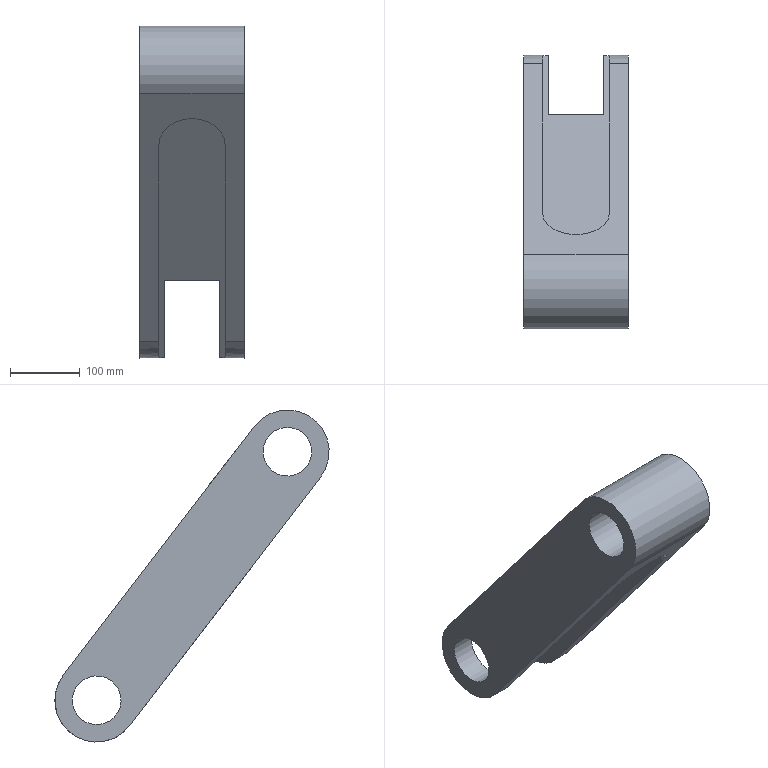Component | NX | LOWER_HYD_ROD | 1 solid | 21 faces | volume 6374617 mm3 | plane 13 | cylinder 8 | commonest cylinder face diameters 120 x3 70 x3 95 x2